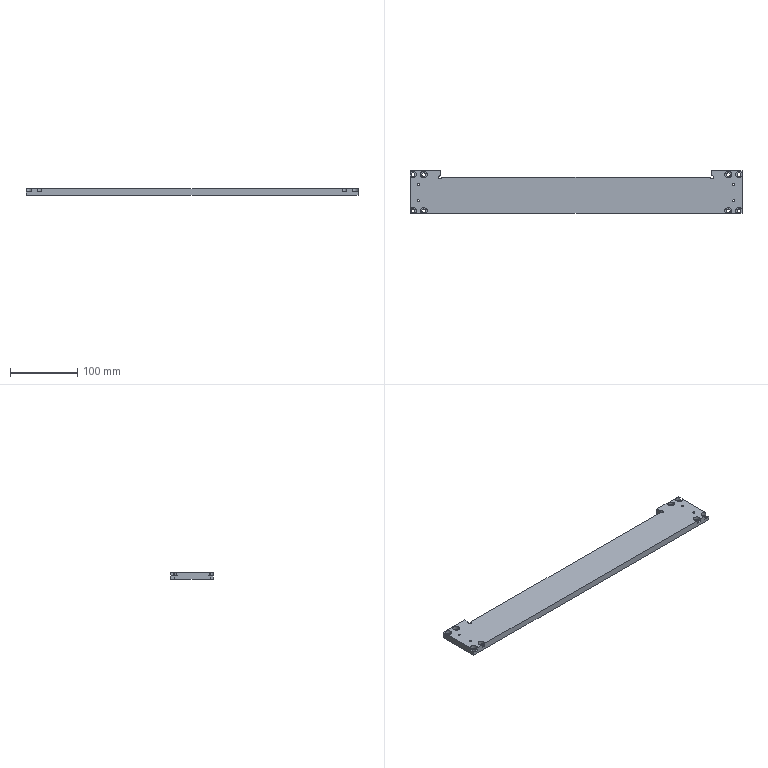Component | SolidWorks | 30-29A-1 | 1 solid | 73 faces | box 495 x 64 x 10 mm | volume 270700 mm3 | cylinder 49 | plane 18 | cone 6 | commonest cylinder face diameters 5.5 x16 10 x16 5 x9 3 x8
build123d program:
from build123d import *

# Parameters (mm, degrees)
SKETCH1_W                                         = 495
SKETCH1_H                                         = 64
EXTRUDE1_DEPTH                                    = 10
M5_SOCKET_HEAD_CAP_SCREW_COUNTERBORE1_D           = 5.5
M5_SOCKET_HEAD_CAP_SCREW_COUNTERBORE1_CBORE_D     = 10
M5_SOCKET_HEAD_CAP_SCREW_COUNTERBORE1_CBORE_DEPTH = 5
SKETCH30_R                                        = 1.5
CUT_EXTRUDE16_DEPTH                               = 10
SKETCH31_W                                        = 405
SKETCH31_H                                        = 10
CUT_EXTRUDE17_DEPTH                               = 10
M6_TAPPED_HOLE1_D                                 = 5
M6_TAPPED_HOLE1_DEPTH                             = 17
M6_TAPPED_HOLE1_TIP                               = 1.502
SKETCH34_R                                        = 2.5
CUT_EXTRUDE18_DEPTH                               = 250.76
CUT_EXTRUDE19_DEPTH                               = 5


with BuildPart() as part:
    # Sketch1 → Extrude1 (new body)
    with BuildSketch(Plane.XY):
        Rectangle(SKETCH1_W, SKETCH1_H)
    extrude(amount=EXTRUDE1_DEPTH)

    # M5 Socket Head Cap Screw Counterbore1 (through all)
    with Locations(Plane.XY.offset(10)):
        with Locations((-227, -28), (-243, -28), (-243, 26), (-227, 26)):
            m5_socket_head_cap_screw_counterbore1 = CounterBoreHole(M5_SOCKET_HEAD_CAP_SCREW_COUNTERBORE1_D / 2, M5_SOCKET_HEAD_CAP_SCREW_COUNTERBORE1_CBORE_D / 2, M5_SOCKET_HEAD_CAP_SCREW_COUNTERBORE1_CBORE_DEPTH)

    # Mirror1: M5 Socket Head Cap Screw Counterbore1 across plane
    add(m5_socket_head_cap_screw_counterbore1.mirror(Plane(origin=(0, 0, 0), x_dir=(0, 0, 1), z_dir=(1, 0, 0))), mode=Mode.SUBTRACT)

    # Sketch30 → Cut-Extrude16 (cut)
    with BuildSketch(Plane.XY.offset(10)):
        with Locations((-235, 11)):
            Circle(SKETCH30_R)
        with Locations((-235, -13)):
            Circle(SKETCH30_R)
        with Locations(Location((235, -13, 0), (0, 0, 180))):
            Circle(SKETCH30_R)
        with Locations(Location((235, 11, 0), (0, 0, 180))):
            Circle(SKETCH30_R)
    extrude(amount=-CUT_EXTRUDE16_DEPTH, mode=Mode.SUBTRACT)

    # Sketch31 → Cut-Extrude17 (cut)
    with BuildSketch(Plane(origin=(0, 32, 0), x_dir=(1, 0, 0), z_dir=(0, 1, 0))):
        with Locations((0, -5)):
            Rectangle(SKETCH31_W, SKETCH31_H)
    extrude(amount=-CUT_EXTRUDE17_DEPTH, mode=Mode.SUBTRACT)

    # M6 Tapped Hole1
    with Locations(Plane(origin=(0, 22, 0), x_dir=(-1, 0, 0), z_dir=(0, 1, 0))):
        with Locations((150, 5), (0, 5), (-150, 5)):
            Hole(M6_TAPPED_HOLE1_D / 2, depth=M6_TAPPED_HOLE1_DEPTH)
            with Locations((0, 0, -(M6_TAPPED_HOLE1_DEPTH + M6_TAPPED_HOLE1_TIP / 2))):  # 118° drill point
                Cone(0, M6_TAPPED_HOLE1_D / 2, M6_TAPPED_HOLE1_TIP, mode=Mode.SUBTRACT)

    # Sketch34 → Cut-Extrude18 (cut, through all)
    with BuildSketch(Plane.XY.offset(10)):
        with Locations((-202.5, 22)):
            Circle(SKETCH34_R)
        with Locations((202.5, 22)):
            Circle(SKETCH34_R)
    extrude(amount=-CUT_EXTRUDE18_DEPTH, mode=Mode.SUBTRACT)

    # Sketch35 → Cut-Extrude19 (cut)
    with BuildSketch(Plane.XY.offset(10)):
        with BuildLine():
            Line((-247.5, -30.179), (-247.5, -32))
            Line((-247.5, -32), (-246, -32))
            ThreePointArc((-246, -32), (-246.859, -31.179), (-247.5, -30.179))
        make_face()
        with BuildLine():
            Line((246, -32), (247.5, -32))
            Line((247.5, -32), (247.5, -30.179))
            ThreePointArc((247.5, -30.179), (246.859, -31.179), (246, -32))
        make_face()
    extrude(amount=-CUT_EXTRUDE19_DEPTH, mode=Mode.SUBTRACT)


solid = part.part

# Placed as in the assembly
solid = solid.moved(Location((-649.208, -5.092, 719.188), (0, 0, 0)))